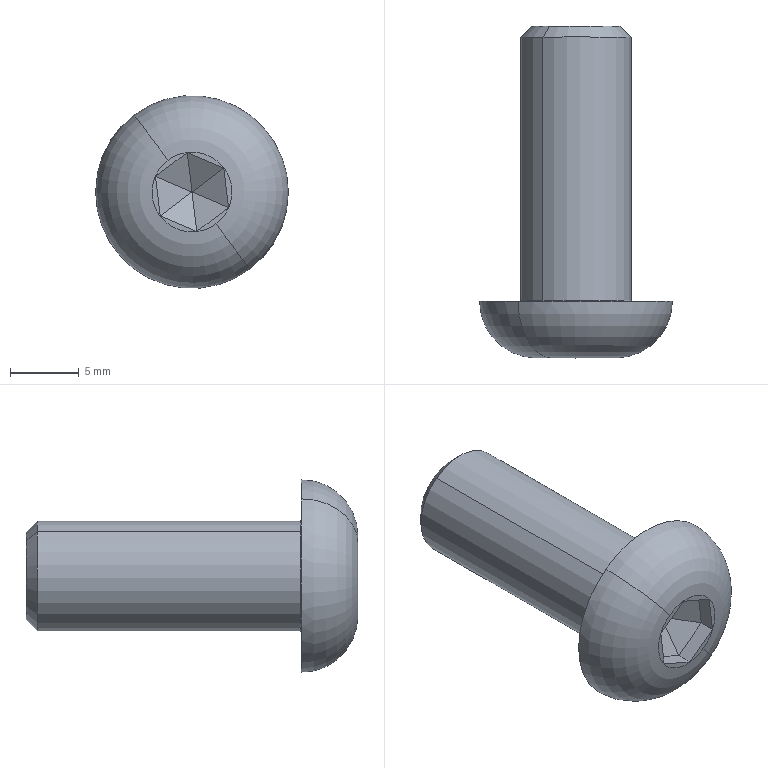Component | SolidWorks | SocketHeadCapScrewM8x20-1 | 1 solid | 24 faces | box 14 x 24.1 x 14 mm | volume 1456 mm3 | plane 16 | torus 4 | cone 2 | cylinder 2 | commonest cylinder face diameters 8 x2 | material Plain Carbon Steel
STEP:
#1=CARTESIAN_POINT('',(1.064,-2.752,9.176));
#2=VERTEX_POINT('',#1);
#3=CARTESIAN_POINT('',(1.257,-2.752,8.917));
#4=VERTEX_POINT('',#3);
#5=CARTESIAN_POINT('',(1.16,-2.752,9.046));
#6=DIRECTION('',(0.,-1.,0.));
#7=DIRECTION('',(0.5999,0.,-0.8));
#8=AXIS2_PLACEMENT_3D('',#5,#6,#7);
#9=CIRCLE('',#8,0.1614);
#10=EDGE_CURVE('',#2,#4,#9,.T.);
#11=ORIENTED_EDGE('',*,*,#10,.F.);
#12=CARTESIAN_POINT('',(1.066,-2.748,9.172));
#13=VERTEX_POINT('',#12);
#14=CARTESIAN_POINT('',(1.064,-2.748,9.176));
#15=DIRECTION('',(0.8,0.,0.5999));
#16=DIRECTION('',(0.5999,0.,-0.8));
#17=AXIS2_PLACEMENT_3D('',#14,#15,#16);
#18=CIRCLE('',#17,0.003937);
#19=EDGE_CURVE('',#2,#13,#18,.T.);
#20=ORIENTED_EDGE('',*,*,#19,.T.);
#21=CARTESIAN_POINT('',(1.255,-2.748,8.92));
#22=VERTEX_POINT('',#21);
#23=CARTESIAN_POINT('',(1.16,-2.748,9.046));
#24=DIRECTION('',(-0.,1.,-0.));
#25=DIRECTION('',(0.5999,0.,-0.8));
#26=AXIS2_PLACEMENT_3D('',#23,#24,#25);
#27=CIRCLE('',#26,0.1575);
#28=EDGE_CURVE('',#22,#13,#27,.T.);
#29=ORIENTED_EDGE('',*,*,#28,.F.);
#30=CARTESIAN_POINT('',(1.257,-2.748,8.917));
#31=DIRECTION('',(-0.8,-0.,-0.5999));
#32=DIRECTION('',(-0.5999,0.,0.8));
#33=AXIS2_PLACEMENT_3D('',#30,#31,#32);
#34=CIRCLE('',#33,0.003937);
#35=EDGE_CURVE('',#4,#22,#34,.T.);
#36=ORIENTED_EDGE('',*,*,#35,.F.);
#37=EDGE_LOOP('',(#11,#20,#29,#36));
#38=FACE_OUTER_BOUND('',#37,.T.);
#39=CARTESIAN_POINT('',(1.16,-2.748,9.046));
#40=DIRECTION('',(0.,-1.,0.));
#41=DIRECTION('',(0.5999,-0.,-0.8));
#42=AXIS2_PLACEMENT_3D('',#39,#40,#41);
#43=TOROIDAL_SURFACE('',#42,0.1614,0.003937);
#44=ADVANCED_FACE('',(#38),#43,.F.);
#45=CARTESIAN_POINT('',(1.085,-1.965,9.147));
#46=VERTEX_POINT('',#45);
#47=CARTESIAN_POINT('',(1.236,-1.965,8.946));
#48=VERTEX_POINT('',#47);
#49=CARTESIAN_POINT('',(1.16,-1.965,9.046));
#50=DIRECTION('',(-0.,1.,-0.));
#51=DIRECTION('',(-0.5999,0.,0.8));
#52=AXIS2_PLACEMENT_3D('',#49,#50,#51);
#53=CIRCLE('',#52,0.126);
#54=EDGE_CURVE('',#46,#48,#53,.T.);
#55=ORIENTED_EDGE('',*,*,#54,.F.);
#56=CARTESIAN_POINT('',(1.066,-1.996,9.172));
#57=VERTEX_POINT('',#56);
#58=CARTESIAN_POINT('',(1.085,-1.965,9.147));
#59=DIRECTION('',(-0.4242,-0.7071,0.5657));
#60=VECTOR('',#59,39.37);
#61=LINE('',#58,#60);
#62=EDGE_CURVE('',#46,#57,#61,.T.);
#63=ORIENTED_EDGE('',*,*,#62,.T.);
#64=CARTESIAN_POINT('',(1.255,-1.996,8.92));
#65=VERTEX_POINT('',#64);
#66=CARTESIAN_POINT('',(1.16,-1.996,9.046));
#67=DIRECTION('',(0.,-1.,0.));
#68=DIRECTION('',(-0.5999,0.,0.8));
#69=AXIS2_PLACEMENT_3D('',#66,#67,#68);
#70=CIRCLE('',#69,0.1575);
#71=EDGE_CURVE('',#65,#57,#70,.T.);
#72=ORIENTED_EDGE('',*,*,#71,.F.);
#73=CARTESIAN_POINT('',(1.236,-1.965,8.946));
#74=DIRECTION('',(0.4242,-0.7071,-0.5657));
#75=VECTOR('',#74,39.37);
#76=LINE('',#73,#75);
#77=EDGE_CURVE('',#48,#65,#76,.T.);
#78=ORIENTED_EDGE('',*,*,#77,.F.);
#79=EDGE_LOOP('',(#55,#63,#72,#78));
#80=FACE_OUTER_BOUND('',#79,.T.);
#81=CARTESIAN_POINT('',(1.16,-1.965,9.046));
#82=DIRECTION('',(0.,-1.,0.));
#83=DIRECTION('',(0.5999,0.,-0.8));
#84=AXIS2_PLACEMENT_3D('',#81,#82,#83);
#85=CONICAL_SURFACE('',#84,0.126,0.7854);
#86=ADVANCED_FACE('',(#80),#85,.T.);
#87=ORIENTED_EDGE('',*,*,#71,.T.);
#88=CARTESIAN_POINT('',(1.066,-1.965,9.172));
#89=DIRECTION('',(0.,-1.,0.));
#90=VECTOR('',#89,39.37);
#91=LINE('',#88,#90);
#92=EDGE_CURVE('',#57,#13,#91,.T.);
#93=ORIENTED_EDGE('',*,*,#92,.T.);
#94=CARTESIAN_POINT('',(1.16,-2.748,9.046));
#95=DIRECTION('',(-0.,1.,-0.));
#96=DIRECTION('',(0.5999,0.,-0.8));
#97=AXIS2_PLACEMENT_3D('',#94,#95,#96);
#98=CIRCLE('',#97,0.1575);
#99=EDGE_CURVE('',#13,#22,#98,.T.);
#100=ORIENTED_EDGE('',*,*,#99,.T.);
#101=CARTESIAN_POINT('',(1.255,-1.965,8.92));
#102=DIRECTION('',(0.,-1.,0.));
#103=VECTOR('',#102,39.37);
#104=LINE('',#101,#103);
#105=EDGE_CURVE('',#65,#22,#104,.T.);
#106=ORIENTED_EDGE('',*,*,#105,.F.);
#107=EDGE_LOOP('',(#87,#93,#100,#106));
#108=FACE_OUTER_BOUND('',#107,.T.);
#109=CARTESIAN_POINT('',(1.16,-1.965,9.046));
#110=DIRECTION('',(0.,-1.,0.));
#111=DIRECTION('',(0.5999,0.,-0.8));
#112=AXIS2_PLACEMENT_3D('',#109,#110,#111);
#113=CYLINDRICAL_SURFACE('',#112,0.1575);
#114=ADVANCED_FACE('',(#108),#113,.T.);
#115=CARTESIAN_POINT('',(1.326,-2.752,8.826));
#116=VERTEX_POINT('',#115);
#117=CARTESIAN_POINT('',(0.9951,-2.752,9.267));
#118=VERTEX_POINT('',#117);
#119=CARTESIAN_POINT('',(1.16,-2.752,9.046));
#120=DIRECTION('',(0.,-1.,0.));
#121=DIRECTION('',(0.5999,0.,-0.8));
#122=AXIS2_PLACEMENT_3D('',#119,#120,#121);
#123=CIRCLE('',#122,0.2756);
#124=EDGE_CURVE('',#116,#118,#123,.T.);
#125=ORIENTED_EDGE('',*,*,#124,.T.);
#126=CARTESIAN_POINT('',(1.092,-2.913,9.138));
#127=VERTEX_POINT('',#126);
#128=CARTESIAN_POINT('',(1.092,-2.752,9.138));
#129=DIRECTION('',(0.8,0.,0.5999));
#130=DIRECTION('',(0.5999,0.,-0.8));
#131=AXIS2_PLACEMENT_3D('',#128,#129,#130);
#132=CIRCLE('',#131,0.1614);
#133=EDGE_CURVE('',#118,#127,#132,.T.);
#134=ORIENTED_EDGE('',*,*,#133,.T.);
#135=CARTESIAN_POINT('',(1.229,-2.913,8.955));
#136=VERTEX_POINT('',#135);
#137=CARTESIAN_POINT('',(1.16,-2.913,9.046));
#138=DIRECTION('',(0.,-1.,0.));
#139=DIRECTION('',(0.5999,0.,-0.8));
#140=AXIS2_PLACEMENT_3D('',#137,#138,#139);
#141=CIRCLE('',#140,0.1142);
#142=EDGE_CURVE('',#136,#127,#141,.T.);
#143=ORIENTED_EDGE('',*,*,#142,.F.);
#144=CARTESIAN_POINT('',(1.229,-2.752,8.955));
#145=DIRECTION('',(-0.8,-0.,-0.5999));
#146=DIRECTION('',(-0.5999,0.,0.8));
#147=AXIS2_PLACEMENT_3D('',#144,#145,#146);
#148=CIRCLE('',#147,0.1614);
#149=EDGE_CURVE('',#116,#136,#148,.T.);
#150=ORIENTED_EDGE('',*,*,#149,.F.);
#151=EDGE_LOOP('',(#125,#134,#143,#150));
#152=FACE_OUTER_BOUND('',#151,.T.);
#153=CARTESIAN_POINT('',(1.16,-2.752,9.046));
#154=DIRECTION('',(0.,-1.,0.));
#155=DIRECTION('',(0.5999,-0.,-0.8));
#156=AXIS2_PLACEMENT_3D('',#153,#154,#155);
#157=TOROIDAL_SURFACE('',#156,0.1142,0.1614);
#158=ADVANCED_FACE('',(#152),#157,.T.);
#159=CARTESIAN_POINT('',(1.16,-2.752,9.046));
#160=DIRECTION('',(0.,-1.,0.));
#161=DIRECTION('',(0.5999,0.,-0.8));
#162=AXIS2_PLACEMENT_3D('',#159,#160,#161);
#163=CIRCLE('',#162,0.1614);
#164=EDGE_CURVE('',#4,#2,#163,.T.);
#165=ORIENTED_EDGE('',*,*,#164,.T.);
#166=ORIENTED_EDGE('',*,*,#10,.T.);
#167=EDGE_LOOP('',(#165,#166));
#168=FACE_BOUND('',#167,.T.);
#169=ORIENTED_EDGE('',*,*,#124,.F.);
#170=CARTESIAN_POINT('',(1.16,-2.752,9.046));
#171=DIRECTION('',(0.,-1.,0.));
#172=DIRECTION('',(0.5999,0.,-0.8));
#173=AXIS2_PLACEMENT_3D('',#170,#171,#172);
#174=CIRCLE('',#173,0.2756);
#175=EDGE_CURVE('',#118,#116,#174,.T.);
#176=ORIENTED_EDGE('',*,*,#175,.F.);
#177=EDGE_LOOP('',(#169,#176));
#178=FACE_OUTER_BOUND('',#177,.T.);
#179=CARTESIAN_POINT('',(1.16,-2.752,9.046));
#180=DIRECTION('',(0.,-1.,0.));
#181=DIRECTION('',(0.5999,-0.,-0.8));
#182=AXIS2_PLACEMENT_3D('',#179,#180,#181);
#183=PLANE('',#182);
#184=ADVANCED_FACE('',(#168,#178),#183,.F.);
#185=CARTESIAN_POINT('',(1.174,-2.913,8.934));
#186=VERTEX_POINT('',#185);
#187=CARTESIAN_POINT('',(1.265,-2.913,9.002));
#188=VERTEX_POINT('',#187);
#189=CARTESIAN_POINT('',(1.174,-2.913,8.934));
#190=DIRECTION('',(0.8,0.,0.5999));
#191=VECTOR('',#190,39.37);
#192=LINE('',#189,#191);
#193=EDGE_CURVE('',#186,#188,#192,.T.);
#194=ORIENTED_EDGE('',*,*,#193,.F.);
#195=CARTESIAN_POINT('',(1.07,-2.913,8.978));
#196=VERTEX_POINT('',#195);
#197=CARTESIAN_POINT('',(1.07,-2.913,8.978));
#198=DIRECTION('',(0.9196,0.,-0.3929));
#199=VECTOR('',#198,39.37);
#200=LINE('',#197,#199);
#201=EDGE_CURVE('',#196,#186,#200,.T.);
#202=ORIENTED_EDGE('',*,*,#201,.F.);
#203=CARTESIAN_POINT('',(1.056,-2.913,9.091));
#204=VERTEX_POINT('',#203);
#205=CARTESIAN_POINT('',(1.056,-2.913,9.091));
#206=DIRECTION('',(0.1195,-0.,-0.9928));
#207=VECTOR('',#206,39.37);
#208=LINE('',#205,#207);
#209=EDGE_CURVE('',#204,#196,#208,.T.);
#210=ORIENTED_EDGE('',*,*,#209,.F.);
#211=CARTESIAN_POINT('',(1.147,-2.913,9.159));
#212=VERTEX_POINT('',#211);
#213=CARTESIAN_POINT('',(1.147,-2.913,9.159));
#214=DIRECTION('',(-0.8,-0.,-0.5999));
#215=VECTOR('',#214,39.37);
#216=LINE('',#213,#215);
#217=EDGE_CURVE('',#212,#204,#216,.T.);
#218=ORIENTED_EDGE('',*,*,#217,.F.);
#219=CARTESIAN_POINT('',(1.251,-2.913,9.115));
#220=VERTEX_POINT('',#219);
#221=CARTESIAN_POINT('',(1.251,-2.913,9.115));
#222=DIRECTION('',(-0.9196,-0.,0.3929));
#223=VECTOR('',#222,39.37);
#224=LINE('',#221,#223);
#225=EDGE_CURVE('',#220,#212,#224,.T.);
#226=ORIENTED_EDGE('',*,*,#225,.F.);
#227=CARTESIAN_POINT('',(1.265,-2.913,9.002));
#228=DIRECTION('',(-0.1195,0.,0.9928));
#229=VECTOR('',#228,39.37);
#230=LINE('',#227,#229);
#231=EDGE_CURVE('',#188,#220,#230,.T.);
#232=ORIENTED_EDGE('',*,*,#231,.F.);
#233=EDGE_LOOP('',(#194,#202,#210,#218,#226,#232));
#234=FACE_BOUND('',#233,.T.);
#235=ORIENTED_EDGE('',*,*,#142,.T.);
#236=CARTESIAN_POINT('',(1.16,-2.913,9.046));
#237=DIRECTION('',(0.,-1.,0.));
#238=DIRECTION('',(0.5999,0.,-0.8));
#239=AXIS2_PLACEMENT_3D('',#236,#237,#238);
#240=CIRCLE('',#239,0.1142);
#241=EDGE_CURVE('',#127,#136,#240,.T.);
#242=ORIENTED_EDGE('',*,*,#241,.T.);
#243=EDGE_LOOP('',(#235,#242));
#244=FACE_OUTER_BOUND('',#243,.T.);
#245=CARTESIAN_POINT('',(1.16,-2.913,9.046));
#246=DIRECTION('',(0.,-1.,0.));
#247=DIRECTION('',(0.5999,-0.,-0.8));
#248=AXIS2_PLACEMENT_3D('',#245,#246,#247);
#249=PLANE('',#248);
#250=ADVANCED_FACE('',(#234,#244),#249,.T.);
#251=ORIENTED_EDGE('',*,*,#133,.F.);
#252=ORIENTED_EDGE('',*,*,#175,.T.);
#253=ORIENTED_EDGE('',*,*,#149,.T.);
#254=ORIENTED_EDGE('',*,*,#241,.F.);
#255=EDGE_LOOP('',(#251,#252,#253,#254));
#256=FACE_OUTER_BOUND('',#255,.T.);
#257=CARTESIAN_POINT('',(1.16,-2.752,9.046));
#258=DIRECTION('',(0.,-1.,0.));
#259=DIRECTION('',(0.5999,-0.,-0.8));
#260=AXIS2_PLACEMENT_3D('',#257,#258,#259);
#261=TOROIDAL_SURFACE('',#260,0.1142,0.1614);
#262=ADVANCED_FACE('',(#256),#261,.T.);
#263=ORIENTED_EDGE('',*,*,#92,.F.);
#264=CARTESIAN_POINT('',(1.16,-1.996,9.046));
#265=DIRECTION('',(0.,-1.,0.));
#266=DIRECTION('',(-0.5999,0.,0.8));
#267=AXIS2_PLACEMENT_3D('',#264,#265,#266);
#268=CIRCLE('',#267,0.1575);
#269=EDGE_CURVE('',#57,#65,#268,.T.);
#270=ORIENTED_EDGE('',*,*,#269,.T.);
#271=ORIENTED_EDGE('',*,*,#105,.T.);
#272=ORIENTED_EDGE('',*,*,#28,.T.);
#273=EDGE_LOOP('',(#263,#270,#271,#272));
#274=FACE_OUTER_BOUND('',#273,.T.);
#275=CARTESIAN_POINT('',(1.16,-1.965,9.046));
#276=DIRECTION('',(0.,-1.,0.));
#277=DIRECTION('',(0.5999,0.,-0.8));
#278=AXIS2_PLACEMENT_3D('',#275,#276,#277);
#279=CYLINDRICAL_SURFACE('',#278,0.1575);
#280=ADVANCED_FACE('',(#274),#279,.T.);
#281=CARTESIAN_POINT('',(1.16,-1.965,9.046));
#282=DIRECTION('',(-0.,1.,-0.));
#283=DIRECTION('',(-0.5999,0.,0.8));
#284=AXIS2_PLACEMENT_3D('',#281,#282,#283);
#285=CIRCLE('',#284,0.126);
#286=EDGE_CURVE('',#48,#46,#285,.T.);
#287=ORIENTED_EDGE('',*,*,#286,.T.);
#288=ORIENTED_EDGE('',*,*,#54,.T.);
#289=EDGE_LOOP('',(#287,#288));
#290=FACE_OUTER_BOUND('',#289,.T.);
#291=CARTESIAN_POINT('',(1.16,-1.965,9.046));
#292=DIRECTION('',(-0.,1.,-0.));
#293=DIRECTION('',(-0.5999,0.,0.8));
#294=AXIS2_PLACEMENT_3D('',#291,#292,#293);
#295=PLANE('',#294);
#296=ADVANCED_FACE('',(#290),#295,.T.);
#297=CARTESIAN_POINT('',(1.265,-2.868,9.002));
#298=VERTEX_POINT('',#297);
#299=CARTESIAN_POINT('',(1.265,-2.811,9.002));
#300=DIRECTION('',(0.,-1.,0.));
#301=VECTOR('',#300,39.37);
#302=LINE('',#299,#301);
#303=EDGE_CURVE('',#298,#188,#302,.T.);
#304=ORIENTED_EDGE('',*,*,#303,.F.);
#305=CARTESIAN_POINT('',(1.174,-2.868,8.934));
#306=VERTEX_POINT('',#305);
#307=CARTESIAN_POINT('',(1.174,-2.868,8.934));
#308=DIRECTION('',(-0.8,-0.,-0.5999));
#309=VECTOR('',#308,39.37);
#310=LINE('',#307,#309);
#311=EDGE_CURVE('',#298,#306,#310,.T.);
#312=ORIENTED_EDGE('',*,*,#311,.T.);
#313=CARTESIAN_POINT('',(1.174,-2.811,8.934));
#314=DIRECTION('',(0.,-1.,0.));
#315=VECTOR('',#314,39.37);
#316=LINE('',#313,#315);
#317=EDGE_CURVE('',#306,#186,#316,.T.);
#318=ORIENTED_EDGE('',*,*,#317,.T.);
#319=ORIENTED_EDGE('',*,*,#193,.T.);
#320=EDGE_LOOP('',(#304,#312,#318,#319));
#321=FACE_OUTER_BOUND('',#320,.T.);
#322=CARTESIAN_POINT('',(1.174,-2.811,8.934));
#323=DIRECTION('',(0.5999,-0.,-0.8));
#324=DIRECTION('',(0.8,0.,0.5999));
#325=AXIS2_PLACEMENT_3D('',#322,#323,#324);
#326=PLANE('',#325);
#327=ADVANCED_FACE('',(#321),#326,.F.);
#328=ORIENTED_EDGE('',*,*,#317,.F.);
#329=CARTESIAN_POINT('',(1.07,-2.868,8.978));
#330=VERTEX_POINT('',#329);
#331=CARTESIAN_POINT('',(1.07,-2.868,8.978));
#332=DIRECTION('',(-0.9196,-0.,0.3929));
#333=VECTOR('',#332,39.37);
#334=LINE('',#331,#333);
#335=EDGE_CURVE('',#306,#330,#334,.T.);
#336=ORIENTED_EDGE('',*,*,#335,.T.);
#337=CARTESIAN_POINT('',(1.07,-2.811,8.978));
#338=DIRECTION('',(0.,-1.,0.));
#339=VECTOR('',#338,39.37);
#340=LINE('',#337,#339);
#341=EDGE_CURVE('',#330,#196,#340,.T.);
#342=ORIENTED_EDGE('',*,*,#341,.T.);
#343=ORIENTED_EDGE('',*,*,#201,.T.);
#344=EDGE_LOOP('',(#328,#336,#342,#343));
#345=FACE_OUTER_BOUND('',#344,.T.);
#346=CARTESIAN_POINT('',(1.07,-2.811,8.978));
#347=DIRECTION('',(-0.3929,-0.,-0.9196));
#348=DIRECTION('',(0.9196,0.,-0.3929));
#349=AXIS2_PLACEMENT_3D('',#346,#347,#348);
#350=PLANE('',#349);
#351=ADVANCED_FACE('',(#345),#350,.F.);
#352=ORIENTED_EDGE('',*,*,#341,.F.);
#353=CARTESIAN_POINT('',(1.056,-2.868,9.091));
#354=VERTEX_POINT('',#353);
#355=CARTESIAN_POINT('',(1.056,-2.868,9.091));
#356=DIRECTION('',(-0.1195,0.,0.9928));
#357=VECTOR('',#356,39.37);
#358=LINE('',#355,#357);
#359=EDGE_CURVE('',#330,#354,#358,.T.);
#360=ORIENTED_EDGE('',*,*,#359,.T.);
#361=CARTESIAN_POINT('',(1.056,-2.811,9.091));
#362=DIRECTION('',(0.,-1.,0.));
#363=VECTOR('',#362,39.37);
#364=LINE('',#361,#363);
#365=EDGE_CURVE('',#354,#204,#364,.T.);
#366=ORIENTED_EDGE('',*,*,#365,.T.);
#367=ORIENTED_EDGE('',*,*,#209,.T.);
#368=EDGE_LOOP('',(#352,#360,#366,#367));
#369=FACE_OUTER_BOUND('',#368,.T.);
#370=CARTESIAN_POINT('',(1.056,-2.811,9.091));
#371=DIRECTION('',(-0.9928,-0.,-0.1195));
#372=DIRECTION('',(0.1195,-0.,-0.9928));
#373=AXIS2_PLACEMENT_3D('',#370,#371,#372);
#374=PLANE('',#373);
#375=ADVANCED_FACE('',(#369),#374,.F.);
#376=ORIENTED_EDGE('',*,*,#365,.F.);
#377=CARTESIAN_POINT('',(1.147,-2.868,9.159));
#378=VERTEX_POINT('',#377);
#379=CARTESIAN_POINT('',(1.147,-2.868,9.159));
#380=DIRECTION('',(0.8,0.,0.5999));
#381=VECTOR('',#380,39.37);
#382=LINE('',#379,#381);
#383=EDGE_CURVE('',#354,#378,#382,.T.);
#384=ORIENTED_EDGE('',*,*,#383,.T.);
#385=CARTESIAN_POINT('',(1.147,-2.811,9.159));
#386=DIRECTION('',(0.,-1.,0.));
#387=VECTOR('',#386,39.37);
#388=LINE('',#385,#387);
#389=EDGE_CURVE('',#378,#212,#388,.T.);
#390=ORIENTED_EDGE('',*,*,#389,.T.);
#391=ORIENTED_EDGE('',*,*,#217,.T.);
#392=EDGE_LOOP('',(#376,#384,#390,#391));
#393=FACE_OUTER_BOUND('',#392,.T.);
#394=CARTESIAN_POINT('',(1.147,-2.811,9.159));
#395=DIRECTION('',(-0.5999,0.,0.8));
#396=DIRECTION('',(0.,-1.,0.));
#397=AXIS2_PLACEMENT_3D('',#394,#395,#396);
#398=PLANE('',#397);
#399=ADVANCED_FACE('',(#393),#398,.F.);
#400=ORIENTED_EDGE('',*,*,#389,.F.);
#401=CARTESIAN_POINT('',(1.251,-2.868,9.115));
#402=VERTEX_POINT('',#401);
#403=CARTESIAN_POINT('',(1.251,-2.868,9.115));
#404=DIRECTION('',(0.9196,0.,-0.3929));
#405=VECTOR('',#404,39.37);
#406=LINE('',#403,#405);
#407=EDGE_CURVE('',#378,#402,#406,.T.);
#408=ORIENTED_EDGE('',*,*,#407,.T.);
#409=CARTESIAN_POINT('',(1.251,-2.811,9.115));
#410=DIRECTION('',(0.,-1.,0.));
#411=VECTOR('',#410,39.37);
#412=LINE('',#409,#411);
#413=EDGE_CURVE('',#402,#220,#412,.T.);
#414=ORIENTED_EDGE('',*,*,#413,.T.);
#415=ORIENTED_EDGE('',*,*,#225,.T.);
#416=EDGE_LOOP('',(#400,#408,#414,#415));
#417=FACE_OUTER_BOUND('',#416,.T.);
#418=CARTESIAN_POINT('',(1.251,-2.811,9.115));
#419=DIRECTION('',(0.3929,0.,0.9196));
#420=DIRECTION('',(-0.9196,-0.,0.3929));
#421=AXIS2_PLACEMENT_3D('',#418,#419,#420);
#422=PLANE('',#421);
#423=ADVANCED_FACE('',(#417),#422,.F.);
#424=ORIENTED_EDGE('',*,*,#413,.F.);
#425=CARTESIAN_POINT('',(1.265,-2.868,9.002));
#426=DIRECTION('',(0.1195,-0.,-0.9928));
#427=VECTOR('',#426,39.37);
#428=LINE('',#425,#427);
#429=EDGE_CURVE('',#402,#298,#428,.T.);
#430=ORIENTED_EDGE('',*,*,#429,.T.);
#431=ORIENTED_EDGE('',*,*,#303,.T.);
#432=ORIENTED_EDGE('',*,*,#231,.T.);
#433=EDGE_LOOP('',(#424,#430,#431,#432));
#434=FACE_OUTER_BOUND('',#433,.T.);
#435=CARTESIAN_POINT('',(1.265,-2.811,9.002));
#436=DIRECTION('',(0.9928,0.,0.1195));
#437=DIRECTION('',(-0.1195,0.,0.9928));
#438=AXIS2_PLACEMENT_3D('',#435,#436,#437);
#439=PLANE('',#438);
#440=ADVANCED_FACE('',(#434),#439,.F.);
#441=CARTESIAN_POINT('',(1.16,-2.811,9.047));
#442=VERTEX_POINT('',#441);
#443=CARTESIAN_POINT('',(1.16,-2.811,9.047));
#444=VERTEX_POINT('',#443);
#445=CARTESIAN_POINT('',(1.16,-2.811,9.047));
#446=DIRECTION('',(-0.8,-0.,-0.5999));
#447=VECTOR('',#446,39.37);
#448=LINE('',#445,#447);
#449=EDGE_CURVE('',#442,#444,#448,.T.);
#450=ORIENTED_EDGE('',*,*,#449,.T.);
#451=CARTESIAN_POINT('',(1.16,-2.811,9.046));
#452=VERTEX_POINT('',#451);
#453=CARTESIAN_POINT('',(1.16,-2.811,9.046));
#454=DIRECTION('',(0.1195,-0.,-0.9928));
#455=VECTOR('',#454,39.37);
#456=LINE('',#453,#455);
#457=EDGE_CURVE('',#444,#452,#456,.T.);
#458=ORIENTED_EDGE('',*,*,#457,.T.);
#459=CARTESIAN_POINT('',(1.16,-2.811,9.046));
#460=VERTEX_POINT('',#459);
#461=CARTESIAN_POINT('',(1.16,-2.811,9.046));
#462=DIRECTION('',(0.9196,0.,-0.3929));
#463=VECTOR('',#462,39.37);
#464=LINE('',#461,#463);
#465=EDGE_CURVE('',#452,#460,#464,.T.);
#466=ORIENTED_EDGE('',*,*,#465,.T.);
#467=CARTESIAN_POINT('',(1.161,-2.811,9.046));
#468=VERTEX_POINT('',#467);
#469=CARTESIAN_POINT('',(1.161,-2.811,9.046));
#470=DIRECTION('',(0.8,0.,0.5999));
#471=VECTOR('',#470,39.37);
#472=LINE('',#469,#471);
#473=EDGE_CURVE('',#460,#468,#472,.T.);
#474=ORIENTED_EDGE('',*,*,#473,.T.);
#475=CARTESIAN_POINT('',(1.161,-2.811,9.047));
#476=VERTEX_POINT('',#475);
#477=CARTESIAN_POINT('',(1.161,-2.811,9.047));
#478=DIRECTION('',(-0.1195,0.,0.9928));
#479=VECTOR('',#478,39.37);
#480=LINE('',#477,#479);
#481=EDGE_CURVE('',#468,#476,#480,.T.);
#482=ORIENTED_EDGE('',*,*,#481,.T.);
#483=CARTESIAN_POINT('',(1.16,-2.811,9.047));
#484=DIRECTION('',(-0.9196,-0.,0.3929));
#485=VECTOR('',#484,39.37);
#486=LINE('',#483,#485);
#487=EDGE_CURVE('',#476,#442,#486,.T.);
#488=ORIENTED_EDGE('',*,*,#487,.T.);
#489=EDGE_LOOP('',(#450,#458,#466,#474,#482,#488));
#490=FACE_OUTER_BOUND('',#489,.T.);
#491=CARTESIAN_POINT('',(1.16,-2.811,9.046));
#492=DIRECTION('',(0.,-1.,0.));
#493=DIRECTION('',(0.5999,-0.,-0.8));
#494=AXIS2_PLACEMENT_3D('',#491,#492,#493);
#495=PLANE('',#494);
#496=ADVANCED_FACE('',(#490),#495,.T.);
#497=ORIENTED_EDGE('',*,*,#62,.F.);
#498=ORIENTED_EDGE('',*,*,#286,.F.);
#499=ORIENTED_EDGE('',*,*,#77,.T.);
#500=ORIENTED_EDGE('',*,*,#269,.F.);
#501=EDGE_LOOP('',(#497,#498,#499,#500));
#502=FACE_OUTER_BOUND('',#501,.T.);
#503=CARTESIAN_POINT('',(1.16,-1.965,9.046));
#504=DIRECTION('',(0.,-1.,0.));
#505=DIRECTION('',(0.5999,0.,-0.8));
#506=AXIS2_PLACEMENT_3D('',#503,#504,#505);
#507=CONICAL_SURFACE('',#506,0.126,0.7854);
#508=ADVANCED_FACE('',(#502),#507,.T.);
#509=CARTESIAN_POINT('',(1.161,-2.811,9.046));
#510=DIRECTION('',(-0.8225,0.4472,0.3514));
#511=VECTOR('',#510,39.37);
#512=LINE('',#509,#511);
#513=EDGE_CURVE('',#298,#468,#512,.T.);
#514=ORIENTED_EDGE('',*,*,#513,.F.);
#515=ORIENTED_EDGE('',*,*,#429,.F.);
#516=CARTESIAN_POINT('',(1.161,-2.811,9.047));
#517=DIRECTION('',(0.7156,-0.4472,0.5366));
#518=VECTOR('',#517,39.37);
#519=LINE('',#516,#518);
#520=EDGE_CURVE('',#476,#402,#519,.T.);
#521=ORIENTED_EDGE('',*,*,#520,.F.);
#522=ORIENTED_EDGE('',*,*,#481,.F.);
#523=EDGE_LOOP('',(#514,#515,#521,#522));
#524=FACE_OUTER_BOUND('',#523,.T.);
#525=CARTESIAN_POINT('',(1.161,-2.811,9.047));
#526=DIRECTION('',(0.4964,0.866,0.05977));
#527=DIRECTION('',(-0.1195,0.,0.9928));
#528=AXIS2_PLACEMENT_3D('',#525,#526,#527);
#529=PLANE('',#528);
#530=ADVANCED_FACE('',(#524),#529,.F.);
#531=ORIENTED_EDGE('',*,*,#520,.T.);
#532=ORIENTED_EDGE('',*,*,#407,.F.);
#533=CARTESIAN_POINT('',(1.16,-2.811,9.047));
#534=DIRECTION('',(-0.1069,-0.4472,0.888));
#535=VECTOR('',#534,39.37);
#536=LINE('',#533,#535);
#537=EDGE_CURVE('',#442,#378,#536,.T.);
#538=ORIENTED_EDGE('',*,*,#537,.F.);
#539=ORIENTED_EDGE('',*,*,#487,.F.);
#540=EDGE_LOOP('',(#531,#532,#538,#539));
#541=FACE_OUTER_BOUND('',#540,.T.);
#542=CARTESIAN_POINT('',(1.16,-2.811,9.047));
#543=DIRECTION('',(0.1964,0.866,0.4598));
#544=DIRECTION('',(-0.9196,-0.,0.3929));
#545=AXIS2_PLACEMENT_3D('',#542,#543,#544);
#546=PLANE('',#545);
#547=ADVANCED_FACE('',(#541),#546,.F.);
#548=ORIENTED_EDGE('',*,*,#513,.T.);
#549=ORIENTED_EDGE('',*,*,#473,.F.);
#550=CARTESIAN_POINT('',(1.16,-2.811,9.046));
#551=DIRECTION('',(-0.1069,0.4472,0.888));
#552=VECTOR('',#551,39.37);
#553=LINE('',#550,#552);
#554=EDGE_CURVE('',#306,#460,#553,.T.);
#555=ORIENTED_EDGE('',*,*,#554,.F.);
#556=ORIENTED_EDGE('',*,*,#311,.F.);
#557=EDGE_LOOP('',(#548,#549,#555,#556));
#558=FACE_OUTER_BOUND('',#557,.T.);
#559=CARTESIAN_POINT('',(1.161,-2.811,9.046));
#560=DIRECTION('',(0.3,0.866,-0.4));
#561=DIRECTION('',(0.8,0.,0.5999));
#562=AXIS2_PLACEMENT_3D('',#559,#560,#561);
#563=PLANE('',#562);
#564=ADVANCED_FACE('',(#558),#563,.F.);
#565=ORIENTED_EDGE('',*,*,#537,.T.);
#566=ORIENTED_EDGE('',*,*,#383,.F.);
#567=CARTESIAN_POINT('',(1.16,-2.811,9.047));
#568=DIRECTION('',(-0.8225,-0.4472,0.3514));
#569=VECTOR('',#568,39.37);
#570=LINE('',#567,#569);
#571=EDGE_CURVE('',#444,#354,#570,.T.);
#572=ORIENTED_EDGE('',*,*,#571,.F.);
#573=ORIENTED_EDGE('',*,*,#449,.F.);
#574=EDGE_LOOP('',(#565,#566,#572,#573));
#575=FACE_OUTER_BOUND('',#574,.T.);
#576=CARTESIAN_POINT('',(1.16,-2.811,9.047));
#577=DIRECTION('',(-0.3,0.866,0.4));
#578=DIRECTION('',(-0.8,-0.,-0.5999));
#579=AXIS2_PLACEMENT_3D('',#576,#577,#578);
#580=PLANE('',#579);
#581=ADVANCED_FACE('',(#575),#580,.F.);
#582=ORIENTED_EDGE('',*,*,#554,.T.);
#583=ORIENTED_EDGE('',*,*,#465,.F.);
#584=CARTESIAN_POINT('',(1.16,-2.811,9.046));
#585=DIRECTION('',(0.7156,0.4472,0.5366));
#586=VECTOR('',#585,39.37);
#587=LINE('',#584,#586);
#588=EDGE_CURVE('',#330,#452,#587,.T.);
#589=ORIENTED_EDGE('',*,*,#588,.F.);
#590=ORIENTED_EDGE('',*,*,#335,.F.);
#591=EDGE_LOOP('',(#582,#583,#589,#590));
#592=FACE_OUTER_BOUND('',#591,.T.);
#593=CARTESIAN_POINT('',(1.16,-2.811,9.046));
#594=DIRECTION('',(-0.1964,0.866,-0.4598));
#595=DIRECTION('',(0.9196,0.,-0.3929));
#596=AXIS2_PLACEMENT_3D('',#593,#594,#595);
#597=PLANE('',#596);
#598=ADVANCED_FACE('',(#592),#597,.F.);
#599=ORIENTED_EDGE('',*,*,#571,.T.);
#600=ORIENTED_EDGE('',*,*,#359,.F.);
#601=ORIENTED_EDGE('',*,*,#588,.T.);
#602=ORIENTED_EDGE('',*,*,#457,.F.);
#603=EDGE_LOOP('',(#599,#600,#601,#602));
#604=FACE_OUTER_BOUND('',#603,.T.);
#605=CARTESIAN_POINT('',(1.16,-2.811,9.046));
#606=DIRECTION('',(-0.4964,0.866,-0.05977));
#607=DIRECTION('',(0.1195,-0.,-0.9928));
#608=AXIS2_PLACEMENT_3D('',#605,#606,#607);
#609=PLANE('',#608);
#610=ADVANCED_FACE('',(#604),#609,.F.);
#611=ORIENTED_EDGE('',*,*,#19,.F.);
#612=ORIENTED_EDGE('',*,*,#164,.F.);
#613=ORIENTED_EDGE('',*,*,#35,.T.);
#614=ORIENTED_EDGE('',*,*,#99,.F.);
#615=EDGE_LOOP('',(#611,#612,#613,#614));
#616=FACE_OUTER_BOUND('',#615,.T.);
#617=CARTESIAN_POINT('',(1.16,-2.748,9.046));
#618=DIRECTION('',(0.,-1.,0.));
#619=DIRECTION('',(0.5999,-0.,-0.8));
#620=AXIS2_PLACEMENT_3D('',#617,#618,#619);
#621=TOROIDAL_SURFACE('',#620,0.1614,0.003937);
#622=ADVANCED_FACE('',(#616),#621,.F.);
#623=CLOSED_SHELL('',(#44,#86,#114,#158,#184,#250,#262,#280,#296,#327,#351,#375,#399,#423,#440,#496,#508,#530,#547,#564,#581,#598,#610,#622));
#624=MANIFOLD_SOLID_BREP('',#623);
#625=CARTESIAN_POINT('',(0.,0.,0.));
#626=DIRECTION('',(0.,0.,1.));
#627=DIRECTION('',(1.,0.,0.));
#628=AXIS2_PLACEMENT_3D('',#625,#626,#627);
#629=(LENGTH_UNIT()NAMED_UNIT(*)SI_UNIT($,.METRE.));
#630=LENGTH_MEASURE_WITH_UNIT(LENGTH_MEASURE(0.0254),#629);
#631=DIMENSIONAL_EXPONENTS(1.,0.,0.,0.,0.,0.,0.);
#632=(CONVERSION_BASED_UNIT('',#630)LENGTH_UNIT()NAMED_UNIT(#631));
#633=UNCERTAINTY_MEASURE_WITH_UNIT(LENGTH_MEASURE(0.00001),#632,'','');
#634=(NAMED_UNIT(*)PLANE_ANGLE_UNIT()SI_UNIT($,.RADIAN.));
#635=(NAMED_UNIT(*)SI_UNIT($,.STERADIAN.)SOLID_ANGLE_UNIT());
#636=(GEOMETRIC_REPRESENTATION_CONTEXT(3)GLOBAL_UNCERTAINTY_ASSIGNED_CONTEXT((#633))GLOBAL_UNIT_ASSIGNED_CONTEXT((#632,#634,#635))REPRESENTATION_CONTEXT('',''));
#637=ADVANCED_BREP_SHAPE_REPRESENTATION('',(#624,#628),#636);
#638=COLOUR_RGB('',0.7922,0.8196,0.9333);
#639=FILL_AREA_STYLE_COLOUR('',#638);
#640=FILL_AREA_STYLE('',(#639));
#641=SURFACE_STYLE_FILL_AREA(#640);
#642=SURFACE_SIDE_STYLE('',(#641));
#643=SURFACE_STYLE_USAGE(.BOTH.,#642);
#644=PRESENTATION_STYLE_ASSIGNMENT((#643));
#645=STYLED_ITEM('',(#644),#624);
#646=PRESENTATION_LAYER_ASSIGNMENT('','',(#645));
#647=(LENGTH_UNIT()NAMED_UNIT(*)SI_UNIT($,.METRE.));
#648=LENGTH_MEASURE_WITH_UNIT(LENGTH_MEASURE(0.0254),#647);
#649=DIMENSIONAL_EXPONENTS(1.,0.,0.,0.,0.,0.,0.);
#650=(CONVERSION_BASED_UNIT('',#648)LENGTH_UNIT()NAMED_UNIT(#649));
#651=UNCERTAINTY_MEASURE_WITH_UNIT(LENGTH_MEASURE(0.00001),#650,'','');
#652=(NAMED_UNIT(*)PLANE_ANGLE_UNIT()SI_UNIT($,.RADIAN.));
#653=(NAMED_UNIT(*)SI_UNIT($,.STERADIAN.)SOLID_ANGLE_UNIT());
#654=(GEOMETRIC_REPRESENTATION_CONTEXT(3)GLOBAL_UNCERTAINTY_ASSIGNED_CONTEXT((#651))GLOBAL_UNIT_ASSIGNED_CONTEXT((#650,#652,#653))REPRESENTATION_CONTEXT('',''));
#655=MECHANICAL_DESIGN_GEOMETRIC_PRESENTATION_REPRESENTATION('',(#645),#654);